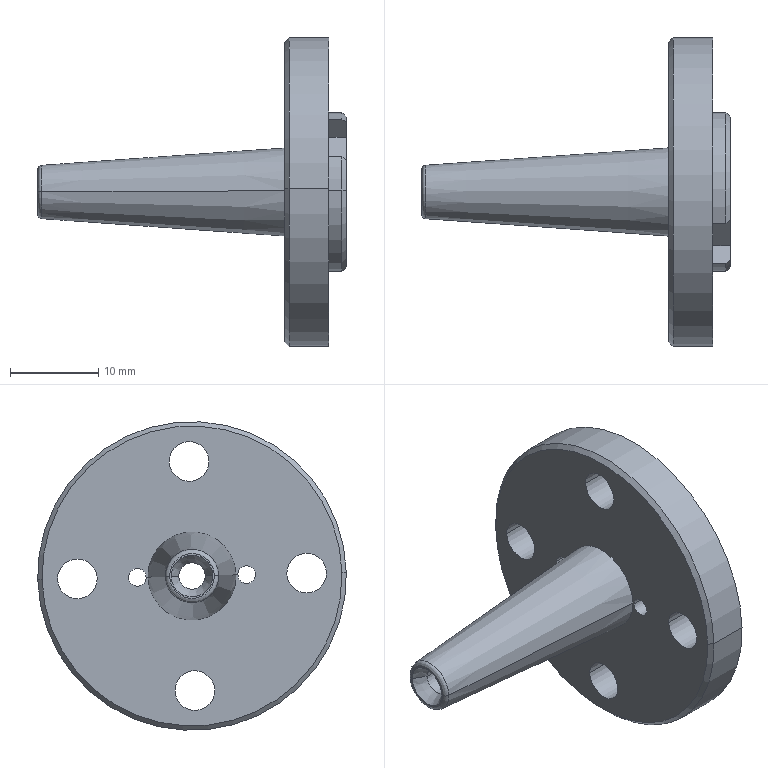Component | SolidWorks | JJDJR-3060-E-007-1 | 1 solid | 39 faces | box 35 x 35 x 35 mm | volume 6073 mm3 | cylinder 19 | cone 11 | plane 7 | torus 2 | commonest cylinder face diameters 4.5 x8 2 x4 18 x3 35 x2 3 x2 | material 40Cr
build123d program:
from build123d import *

# Parameters (mm, degrees)
SKETCH2_2_R                   = 2.25
CUT_EXTRUDE1_DEPTH            = 38.37
FILLET1_R                     = 0.5
CHAMFER1_SIZE                 = 1.5
CHAMFER1_SIZE2                = 0.866
CHAMFER2_SIZE                 = 0.5
SKETCH3_R                     = 1
CUT_EXTRUDE2_DEPTH            = 38.37
CHAMFER3_SIZE                 = 1
CHAMFER4_SIZE                 = 0.5
KEY_RELIEF_NOTCH_REPAIR_DEPTH = 3


with BuildPart() as part:
    # Sketch1_2 → Revolve1 (revolve)
    with BuildSketch(Plane.XY, mode=Mode.PRIVATE) as revolve1_sk:
        Polygon((0, 1.5), (36, 1.5), (36, 3), (8, 5), (8, 17.5), (3, 17.5), (3, 9), (0, 9), align=None)
    revolve(revolve1_sk.sketch.rotate(Axis((0, 0, 0), (1, 0, 0)), 90), axis=Axis((0, 0, 0), (1, 0, 0)))

    # Sketch2_2 → Cut-Extrude1 (cut, through all)
    with BuildSketch(Plane(origin=(8, 0, 0), x_dir=(0, 0, -1), z_dir=(1, 0, 0))):
        with Locations((0, 13)):
            Circle(SKETCH2_2_R)
        with Locations((0, -13)):
            Circle(SKETCH2_2_R)
        with Locations((-13, 0)):
            Circle(SKETCH2_2_R)
        with Locations((13, 0)):
            Circle(SKETCH2_2_R)
    extrude(amount=-CUT_EXTRUDE1_DEPTH, mode=Mode.SUBTRACT)

    # Fillet1
    fillet1_edges = [part.edges().sort_by_distance(p)[0] for p in [
        (36, 0, -3),
    ]]
    fillet(fillet1_edges, radius=FILLET1_R)

    # Chamfer1
    chamfer1_edges = [part.edges().sort_by_distance(p)[0] for p in [
        (36, 0, -1.5),
    ]]
    chamfer1_side = [part.faces().sort_by_distance(p)[0] for p in [
        (18, 0, -1.5),
    ]]
    chamfer(chamfer1_edges, length=CHAMFER1_SIZE, length2=CHAMFER1_SIZE2, reference=chamfer1_side[0])

    # Chamfer2
    chamfer2_edges = [part.edges().sort_by_distance(p)[0] for p in [
        (8, 0, -17.5),
    ]]
    chamfer(chamfer2_edges, length=CHAMFER2_SIZE)

    # Sketch3 → Cut-Extrude2 (cut, through all)
    with BuildSketch(Plane.ZY.offset(-8)):
        with Locations((6.2, 0)):
            Circle(SKETCH3_R)
    cut_extrude2 = extrude(amount=CUT_EXTRUDE2_DEPTH, mode=Mode.SUBTRACT)

    # Mirror1: Cut-Extrude2 across plane
    add(cut_extrude2.mirror(Plane.XY), mode=Mode.SUBTRACT)

    # Chamfer3
    chamfer3_edges = [part.edges().sort_by_distance(p)[0] for p in [
        (0, 0, -1.5),
    ]]
    chamfer(chamfer3_edges, length=CHAMFER3_SIZE)

    # Chamfer4
    chamfer4_edges = [part.edges().sort_by_distance(p)[0] for p in [
        (0, 0, -9),
    ]]
    chamfer(chamfer4_edges, length=CHAMFER4_SIZE)

    # Sketch1 → Spigot face-back 1mm _repair (revolve, cut)
    with BuildSketch(Plane.XY, mode=Mode.PRIVATE) as spigot_face_back_1mm_repair_sk:
        Polygon((-1, 0.5), (-1, 10), (1.5, 10), (1.5, 9), (1, 8.5), (1, 2.5), (2, 1.5), (2, 0.5), align=None)
    revolve(spigot_face_back_1mm_repair_sk.sketch.rotate(Axis((-5, 0, 0), (1, 0, 0)), 90), axis=Axis((-5, 0, 0), (1, 0, 0)), mode=Mode.SUBTRACT)

    # Sketch2 → Key relief notch _repair (cut)
    with BuildSketch(Plane(origin=(0, 0, 0), x_dir=(0, 0, -1), z_dir=(1, 0, 0))):
        Polygon((6.152, 1.768), (9.617, 5.233), (5.233, 9.617), (1.768, 6.152), align=None)
    extrude(amount=KEY_RELIEF_NOTCH_REPAIR_DEPTH, mode=Mode.SUBTRACT)


solid = part.part

# Placed as in the assembly
solid = solid.moved(Location((-137.59, -29.263, -16.52), (-91.43, 0, 180)))